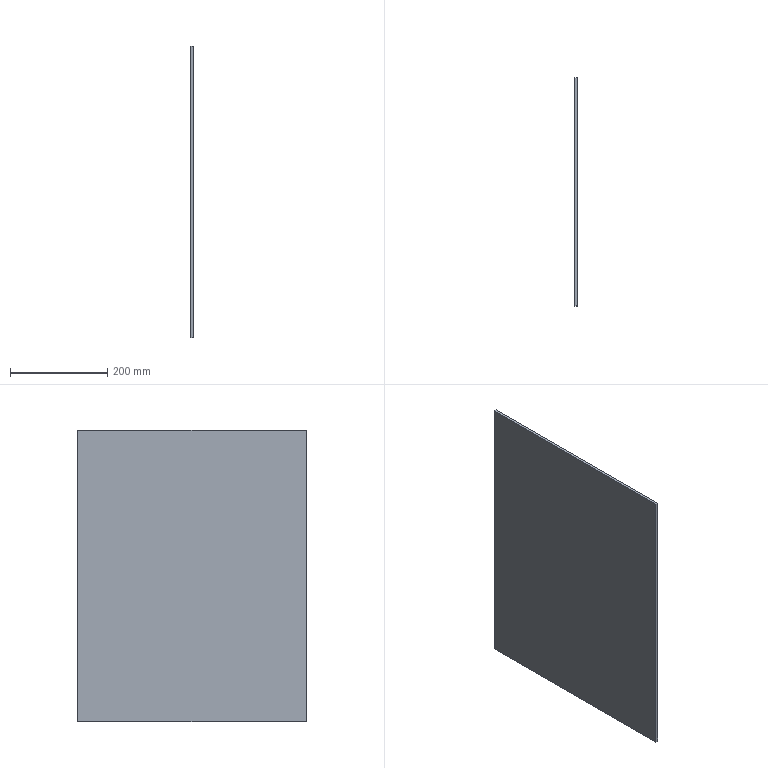Component | SolidWorks | CoverPlate2-1 | 1 solid | 6 faces | box 5 x 470 x 600 mm | volume 1410000 mm3 | plane 6
build123d program:
from build123d import *

# Parameters (mm, degrees)
SKETCH1_W      = 470
SKETCH1_H      = 600
EXTRUDE1_DEPTH = 5


with BuildPart() as part:
    # Sketch1 → Extrude1 (new body)
    with BuildSketch(Plane.XY):
        Rectangle(SKETCH1_W, SKETCH1_H)
    extrude(amount=EXTRUDE1_DEPTH)


solid = part.part

# Placed as in the assembly
solid = solid.moved(Location((320, 375, 280), (90, -90, 0)))
STEP:
#1=COLOUR_RGB('',0.7922,0.8196,0.9333);
#2=FILL_AREA_STYLE_COLOUR('',#1);
#3=FILL_AREA_STYLE('',(#2));
#4=SURFACE_STYLE_FILL_AREA(#3);
#5=SURFACE_SIDE_STYLE('',(#4));
#6=SURFACE_STYLE_USAGE(.BOTH.,#5);
#7=PRESENTATION_STYLE_ASSIGNMENT((#6));
#8=CARTESIAN_POINT('',(12.402,24.016,-0.7874));
#9=VERTEX_POINT('',#8);
#10=CARTESIAN_POINT('',(12.402,24.016,22.835));
#11=VERTEX_POINT('',#10);
#12=CARTESIAN_POINT('',(12.402,24.016,22.835));
#13=DIRECTION('',(0.,-0.,1.));
#14=VECTOR('',#13,39.37);
#15=LINE('',#12,#14);
#16=EDGE_CURVE('',#9,#11,#15,.T.);
#17=ORIENTED_EDGE('',*,*,#16,.T.);
#18=CARTESIAN_POINT('',(12.598,24.016,22.835));
#19=VERTEX_POINT('',#18);
#20=CARTESIAN_POINT('',(12.598,24.016,22.835));
#21=DIRECTION('',(-1.,-0.,0.));
#22=VECTOR('',#21,39.37);
#23=LINE('',#20,#22);
#24=EDGE_CURVE('',#19,#11,#23,.T.);
#25=ORIENTED_EDGE('',*,*,#24,.F.);
#26=CARTESIAN_POINT('',(12.598,24.016,-0.7874));
#27=VERTEX_POINT('',#26);
#28=CARTESIAN_POINT('',(12.598,24.016,22.835));
#29=DIRECTION('',(0.,-0.,1.));
#30=VECTOR('',#29,39.37);
#31=LINE('',#28,#30);
#32=EDGE_CURVE('',#27,#19,#31,.T.);
#33=ORIENTED_EDGE('',*,*,#32,.F.);
#34=CARTESIAN_POINT('',(12.598,24.016,-0.7874));
#35=DIRECTION('',(-1.,-0.,0.));
#36=VECTOR('',#35,39.37);
#37=LINE('',#34,#36);
#38=EDGE_CURVE('',#27,#9,#37,.T.);
#39=ORIENTED_EDGE('',*,*,#38,.T.);
#40=EDGE_LOOP('',(#17,#25,#33,#39));
#41=FACE_OUTER_BOUND('',#40,.T.);
#42=CARTESIAN_POINT('',(12.598,24.016,22.835));
#43=DIRECTION('',(0.,-1.,-0.));
#44=DIRECTION('',(-0.,0.,-1.));
#45=AXIS2_PLACEMENT_3D('',#42,#43,#44);
#46=PLANE('',#45);
#47=ADVANCED_FACE('',(#41),#46,.F.);
#48=CARTESIAN_POINT('',(12.402,5.512,22.835));
#49=VERTEX_POINT('',#48);
#50=CARTESIAN_POINT('',(12.402,5.512,22.835));
#51=DIRECTION('',(0.,-1.,0.));
#52=VECTOR('',#51,39.37);
#53=LINE('',#50,#52);
#54=EDGE_CURVE('',#11,#49,#53,.T.);
#55=ORIENTED_EDGE('',*,*,#54,.T.);
#56=CARTESIAN_POINT('',(12.598,5.512,22.835));
#57=VERTEX_POINT('',#56);
#58=CARTESIAN_POINT('',(12.598,5.512,22.835));
#59=DIRECTION('',(-1.,-0.,0.));
#60=VECTOR('',#59,39.37);
#61=LINE('',#58,#60);
#62=EDGE_CURVE('',#57,#49,#61,.T.);
#63=ORIENTED_EDGE('',*,*,#62,.F.);
#64=CARTESIAN_POINT('',(12.598,5.512,22.835));
#65=DIRECTION('',(0.,-1.,0.));
#66=VECTOR('',#65,39.37);
#67=LINE('',#64,#66);
#68=EDGE_CURVE('',#19,#57,#67,.T.);
#69=ORIENTED_EDGE('',*,*,#68,.F.);
#70=ORIENTED_EDGE('',*,*,#24,.T.);
#71=EDGE_LOOP('',(#55,#63,#69,#70));
#72=FACE_OUTER_BOUND('',#71,.T.);
#73=CARTESIAN_POINT('',(12.598,5.512,22.835));
#74=DIRECTION('',(-0.,-0.,-1.));
#75=DIRECTION('',(-1.,-0.,0.));
#76=AXIS2_PLACEMENT_3D('',#73,#74,#75);
#77=PLANE('',#76);
#78=ADVANCED_FACE('',(#72),#77,.F.);
#79=CARTESIAN_POINT('',(12.402,5.512,-0.7874));
#80=VERTEX_POINT('',#79);
#81=CARTESIAN_POINT('',(12.402,5.512,22.835));
#82=DIRECTION('',(-0.,0.,-1.));
#83=VECTOR('',#82,39.37);
#84=LINE('',#81,#83);
#85=EDGE_CURVE('',#49,#80,#84,.T.);
#86=ORIENTED_EDGE('',*,*,#85,.T.);
#87=CARTESIAN_POINT('',(12.598,5.512,-0.7874));
#88=VERTEX_POINT('',#87);
#89=CARTESIAN_POINT('',(12.598,5.512,-0.7874));
#90=DIRECTION('',(-1.,-0.,0.));
#91=VECTOR('',#90,39.37);
#92=LINE('',#89,#91);
#93=EDGE_CURVE('',#88,#80,#92,.T.);
#94=ORIENTED_EDGE('',*,*,#93,.F.);
#95=CARTESIAN_POINT('',(12.598,5.512,22.835));
#96=DIRECTION('',(-0.,0.,-1.));
#97=VECTOR('',#96,39.37);
#98=LINE('',#95,#97);
#99=EDGE_CURVE('',#57,#88,#98,.T.);
#100=ORIENTED_EDGE('',*,*,#99,.F.);
#101=ORIENTED_EDGE('',*,*,#62,.T.);
#102=EDGE_LOOP('',(#86,#94,#100,#101));
#103=FACE_OUTER_BOUND('',#102,.T.);
#104=CARTESIAN_POINT('',(12.598,5.512,22.835));
#105=DIRECTION('',(-0.,1.,0.));
#106=DIRECTION('',(0.,-0.,1.));
#107=AXIS2_PLACEMENT_3D('',#104,#105,#106);
#108=PLANE('',#107);
#109=ADVANCED_FACE('',(#103),#108,.F.);
#110=CARTESIAN_POINT('',(12.402,5.512,-0.7874));
#111=DIRECTION('',(-0.,1.,-0.));
#112=VECTOR('',#111,39.37);
#113=LINE('',#110,#112);
#114=EDGE_CURVE('',#80,#9,#113,.T.);
#115=ORIENTED_EDGE('',*,*,#114,.T.);
#116=ORIENTED_EDGE('',*,*,#38,.F.);
#117=CARTESIAN_POINT('',(12.598,5.512,-0.7874));
#118=DIRECTION('',(-0.,1.,-0.));
#119=VECTOR('',#118,39.37);
#120=LINE('',#117,#119);
#121=EDGE_CURVE('',#88,#27,#120,.T.);
#122=ORIENTED_EDGE('',*,*,#121,.F.);
#123=ORIENTED_EDGE('',*,*,#93,.T.);
#124=EDGE_LOOP('',(#115,#116,#122,#123));
#125=FACE_OUTER_BOUND('',#124,.T.);
#126=CARTESIAN_POINT('',(12.598,5.512,-0.7874));
#127=DIRECTION('',(0.,0.,1.));
#128=DIRECTION('',(1.,0.,-0.));
#129=AXIS2_PLACEMENT_3D('',#126,#127,#128);
#130=PLANE('',#129);
#131=ADVANCED_FACE('',(#125),#130,.F.);
#132=ORIENTED_EDGE('',*,*,#32,.T.);
#133=ORIENTED_EDGE('',*,*,#68,.T.);
#134=ORIENTED_EDGE('',*,*,#99,.T.);
#135=ORIENTED_EDGE('',*,*,#121,.T.);
#136=EDGE_LOOP('',(#132,#133,#134,#135));
#137=FACE_OUTER_BOUND('',#136,.T.);
#138=CARTESIAN_POINT('',(12.598,14.764,11.024));
#139=DIRECTION('',(1.,0.,-0.));
#140=DIRECTION('',(-0.,1.,-0.));
#141=AXIS2_PLACEMENT_3D('',#138,#139,#140);
#142=PLANE('',#141);
#143=ADVANCED_FACE('',(#137),#142,.T.);
#144=ORIENTED_EDGE('',*,*,#16,.F.);
#145=ORIENTED_EDGE('',*,*,#114,.F.);
#146=ORIENTED_EDGE('',*,*,#85,.F.);
#147=ORIENTED_EDGE('',*,*,#54,.F.);
#148=EDGE_LOOP('',(#144,#145,#146,#147));
#149=FACE_OUTER_BOUND('',#148,.T.);
#150=CARTESIAN_POINT('',(12.402,14.764,11.024));
#151=DIRECTION('',(1.,0.,-0.));
#152=DIRECTION('',(-0.,1.,-0.));
#153=AXIS2_PLACEMENT_3D('',#150,#151,#152);
#154=PLANE('',#153);
#155=ADVANCED_FACE('',(#149),#154,.F.);
#156=CLOSED_SHELL('',(#47,#78,#109,#131,#143,#155));
#157=MANIFOLD_SOLID_BREP('',#156);
#158=STYLED_ITEM('',(#7),#157);
#159=(LENGTH_UNIT()NAMED_UNIT(*)SI_UNIT($,.METRE.));
#160=LENGTH_MEASURE_WITH_UNIT(LENGTH_MEASURE(0.0254),#159);
#161=DIMENSIONAL_EXPONENTS(1.,0.,0.,0.,0.,0.,0.);
#162=(CONVERSION_BASED_UNIT('',#160)LENGTH_UNIT()NAMED_UNIT(#161));
#163=UNCERTAINTY_MEASURE_WITH_UNIT(LENGTH_MEASURE(0.00001),#162,'','');
#164=(NAMED_UNIT(*)PLANE_ANGLE_UNIT()SI_UNIT($,.RADIAN.));
#165=(NAMED_UNIT(*)SI_UNIT($,.STERADIAN.)SOLID_ANGLE_UNIT());
#166=(GEOMETRIC_REPRESENTATION_CONTEXT(3)GLOBAL_UNCERTAINTY_ASSIGNED_CONTEXT((#163))GLOBAL_UNIT_ASSIGNED_CONTEXT((#162,#164,#165))REPRESENTATION_CONTEXT('',''));
#167=MECHANICAL_DESIGN_GEOMETRIC_PRESENTATION_REPRESENTATION('',(#158),#166);
#168=CARTESIAN_POINT('',(0.,0.,0.));
#169=DIRECTION('',(0.,0.,1.));
#170=DIRECTION('',(1.,0.,0.));
#171=AXIS2_PLACEMENT_3D('',#168,#169,#170);
#172=(LENGTH_UNIT()NAMED_UNIT(*)SI_UNIT($,.METRE.));
#173=LENGTH_MEASURE_WITH_UNIT(LENGTH_MEASURE(0.0254),#172);
#174=DIMENSIONAL_EXPONENTS(1.,0.,0.,0.,0.,0.,0.);
#175=(CONVERSION_BASED_UNIT('',#173)LENGTH_UNIT()NAMED_UNIT(#174));
#176=UNCERTAINTY_MEASURE_WITH_UNIT(LENGTH_MEASURE(0.00001),#175,'','');
#177=(NAMED_UNIT(*)PLANE_ANGLE_UNIT()SI_UNIT($,.RADIAN.));
#178=(NAMED_UNIT(*)SI_UNIT($,.STERADIAN.)SOLID_ANGLE_UNIT());
#179=(GEOMETRIC_REPRESENTATION_CONTEXT(3)GLOBAL_UNCERTAINTY_ASSIGNED_CONTEXT((#176))GLOBAL_UNIT_ASSIGNED_CONTEXT((#175,#177,#178))REPRESENTATION_CONTEXT('',''));
#180=ADVANCED_BREP_SHAPE_REPRESENTATION('',(#157,#171),#179);
#181=PRESENTATION_LAYER_ASSIGNMENT('','',(#158));